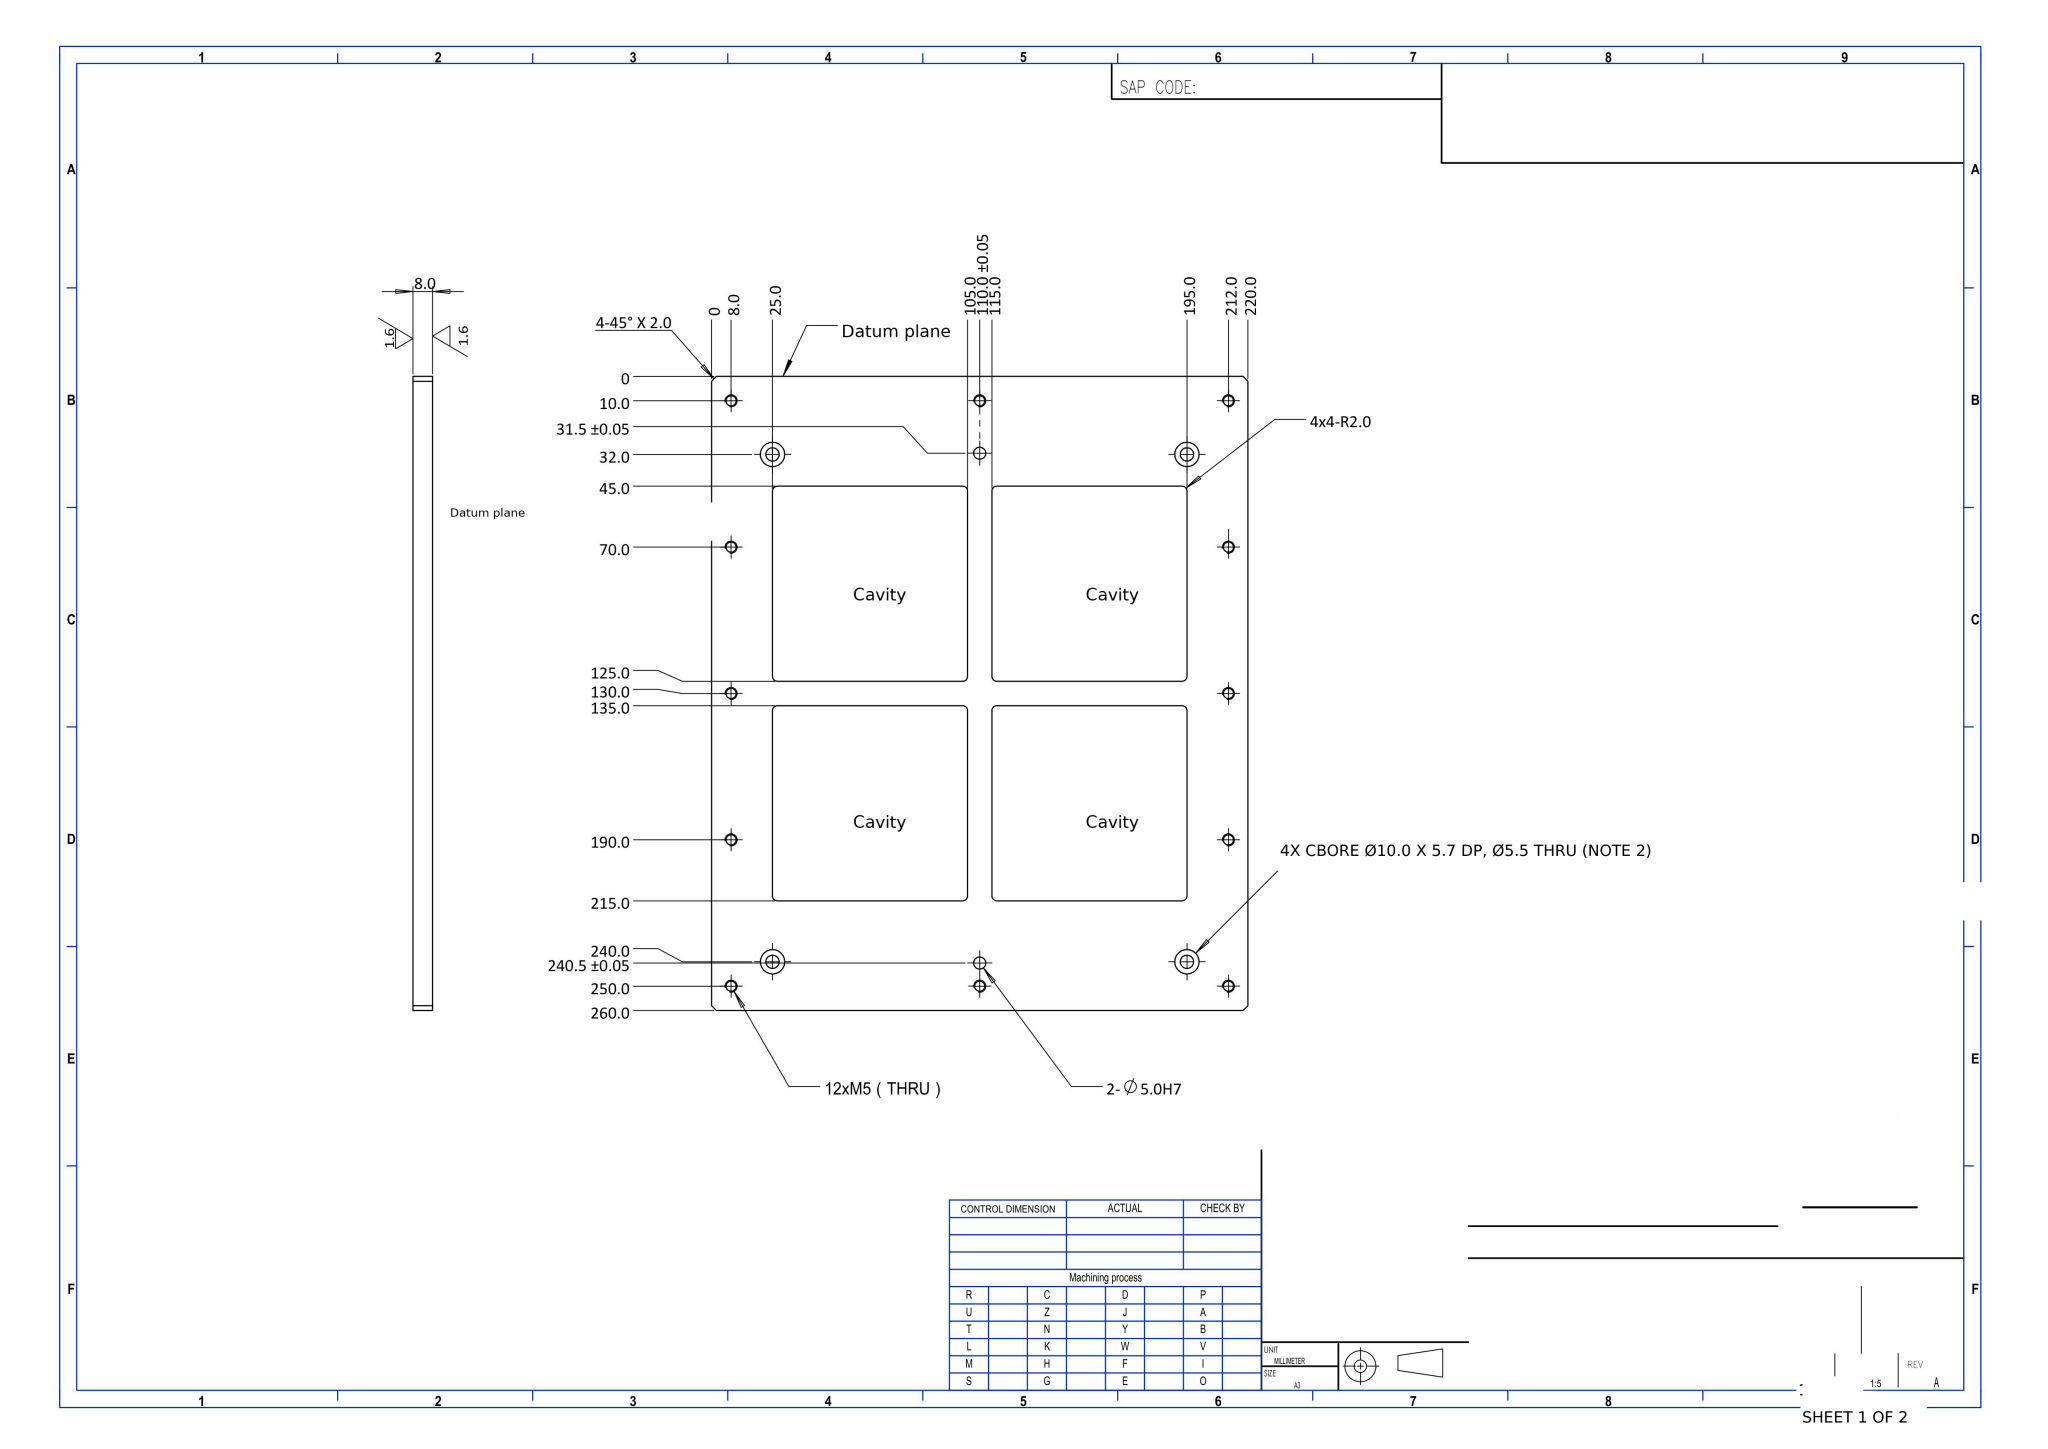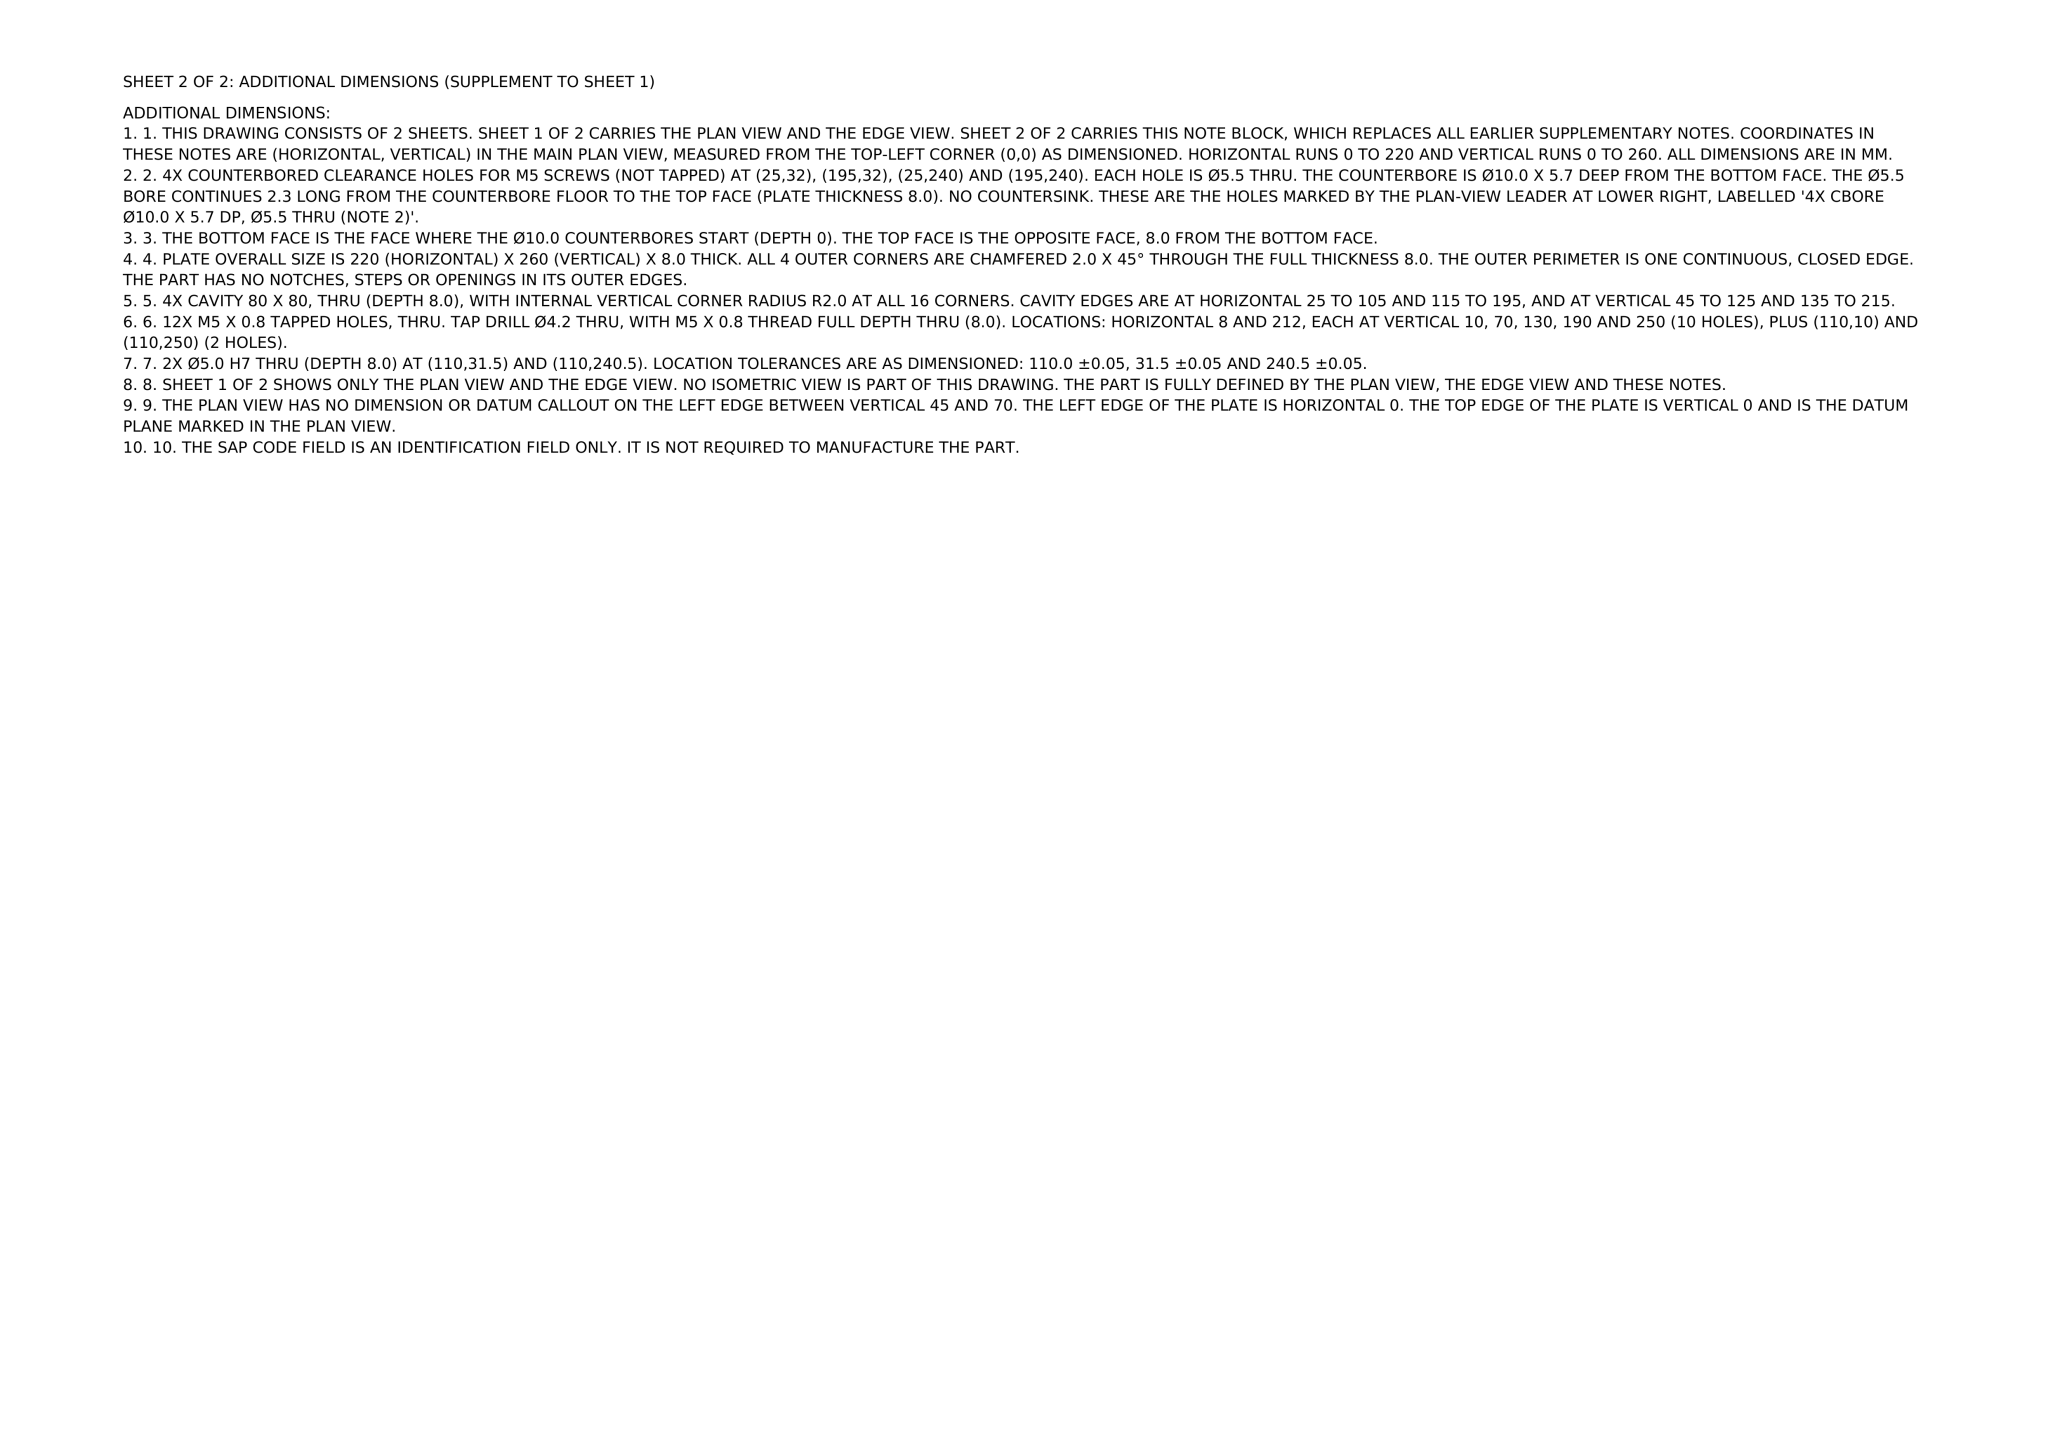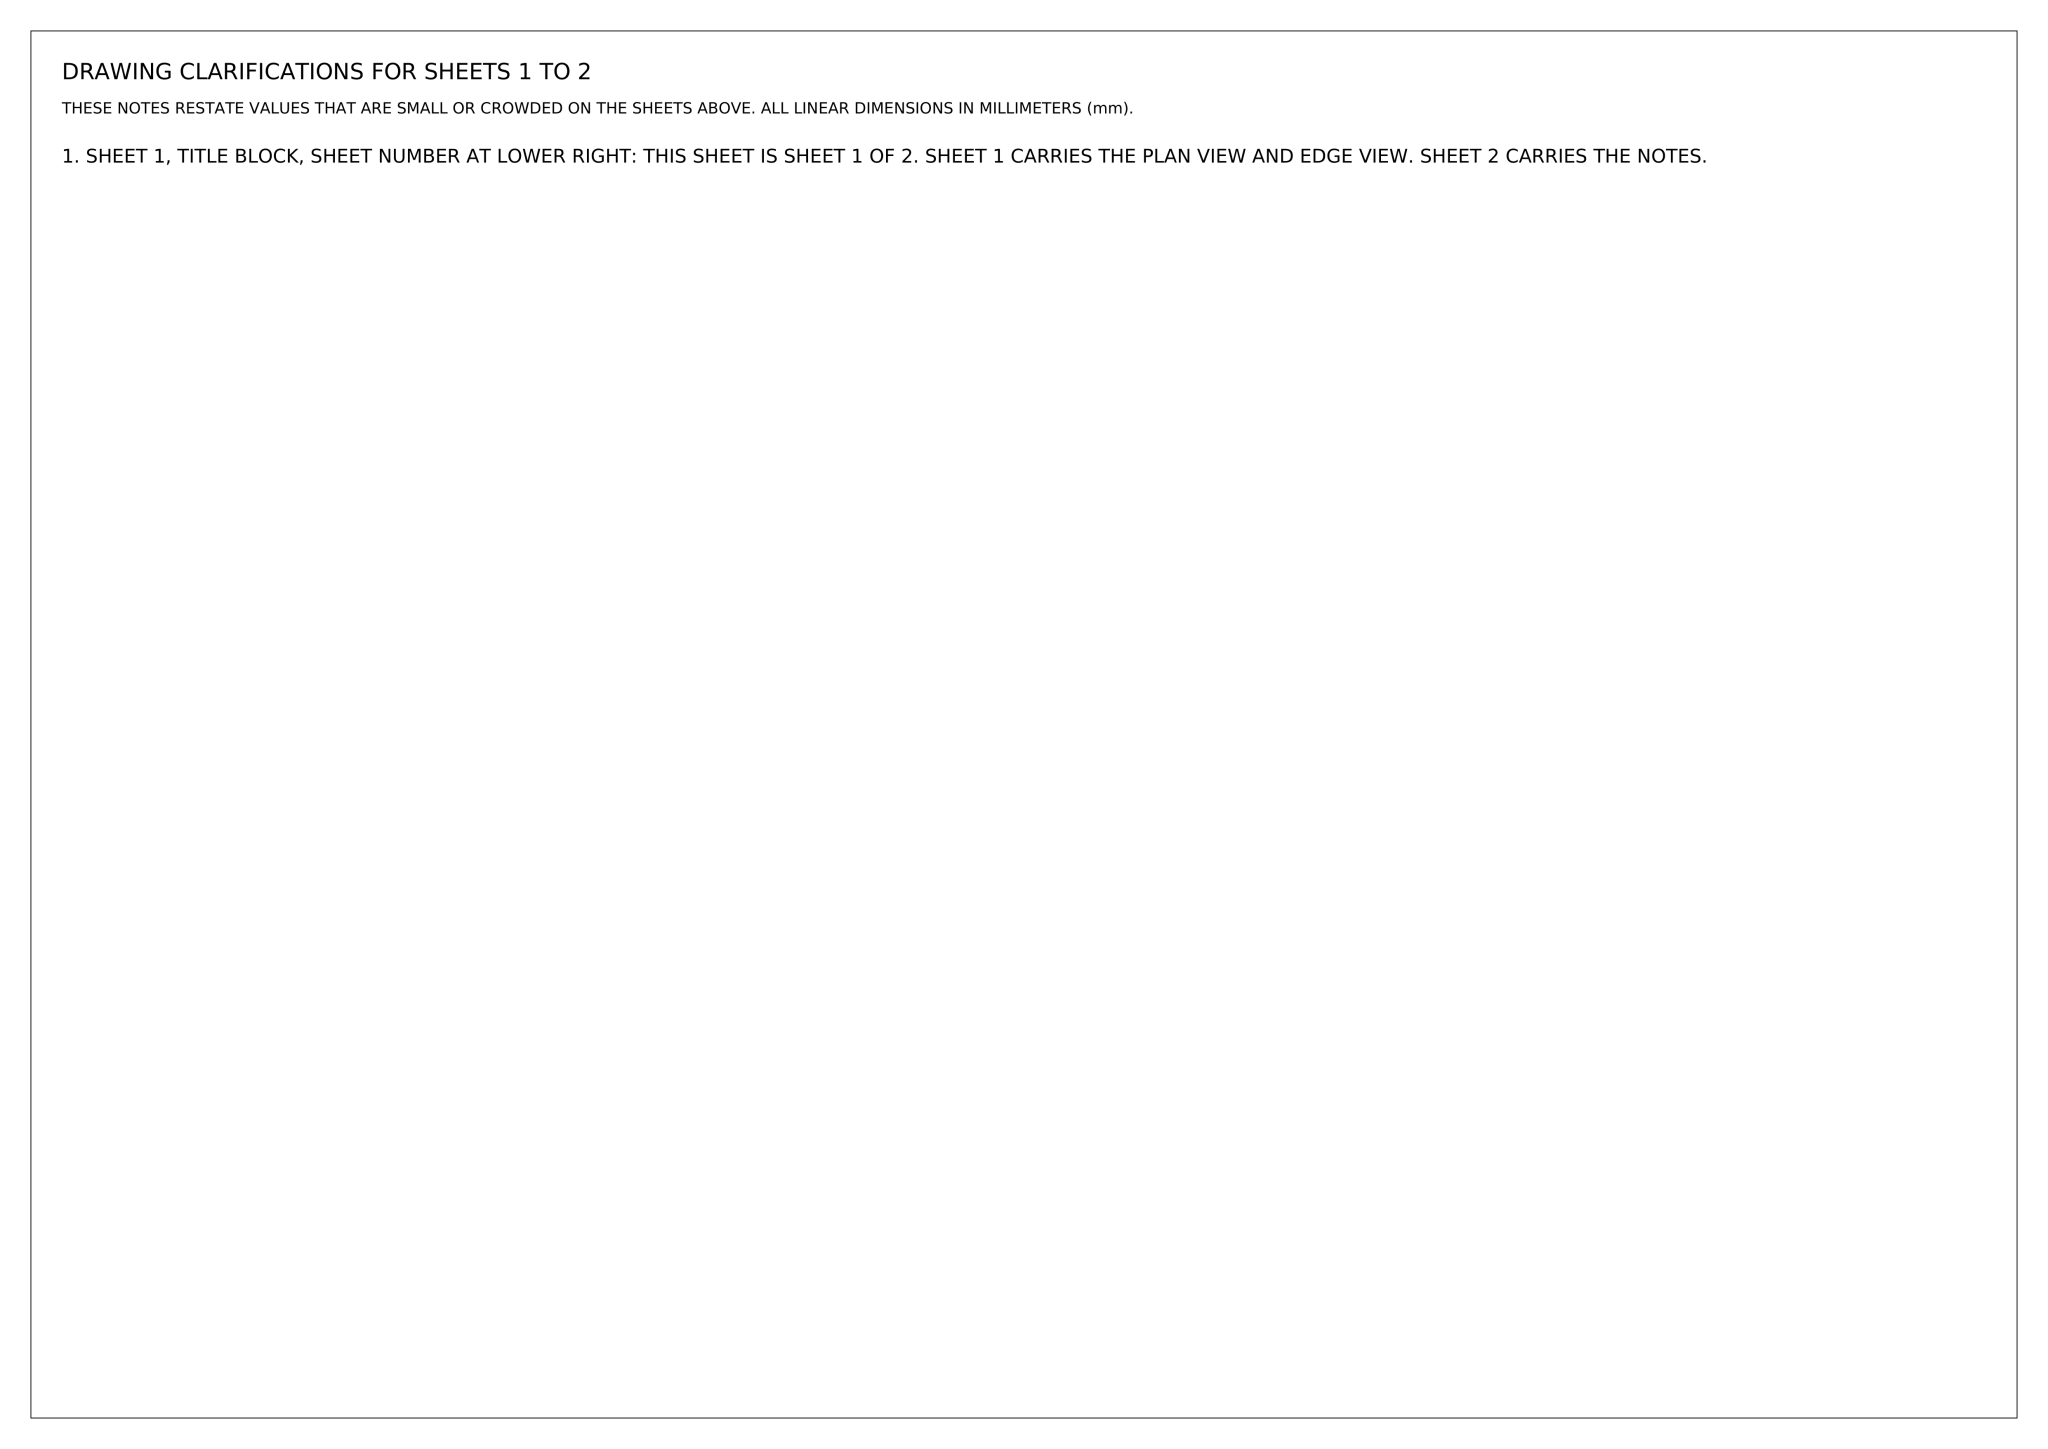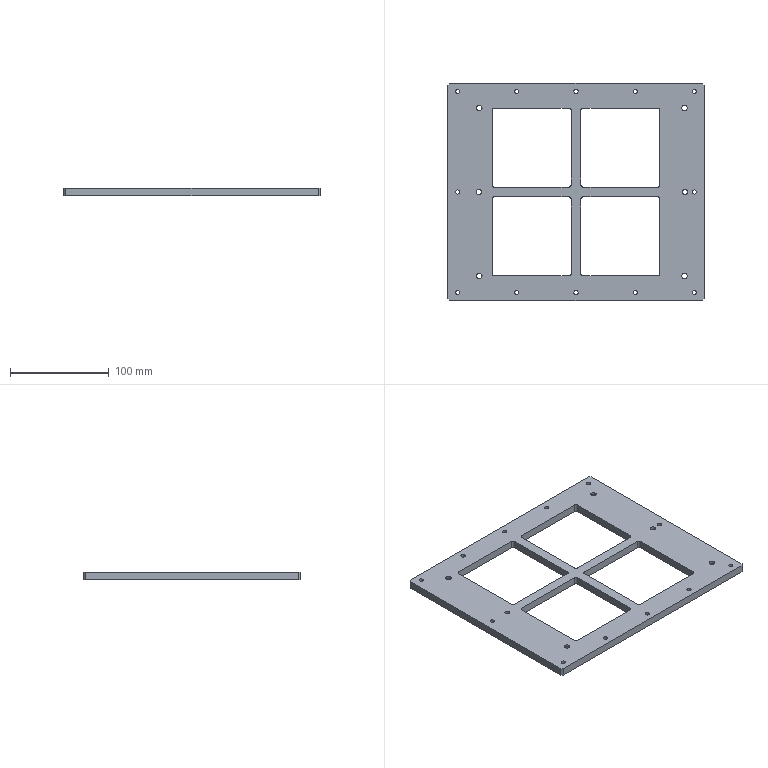Part | NX | mm | 1 solid | 90 faces | box 260 x 220 x 8 mm | volume 249192 mm3 | cylinder 60 | plane 30 | commonest cylinder face diameters 4.2 x24 4 x16 10 x8 5.5 x8 5 x4